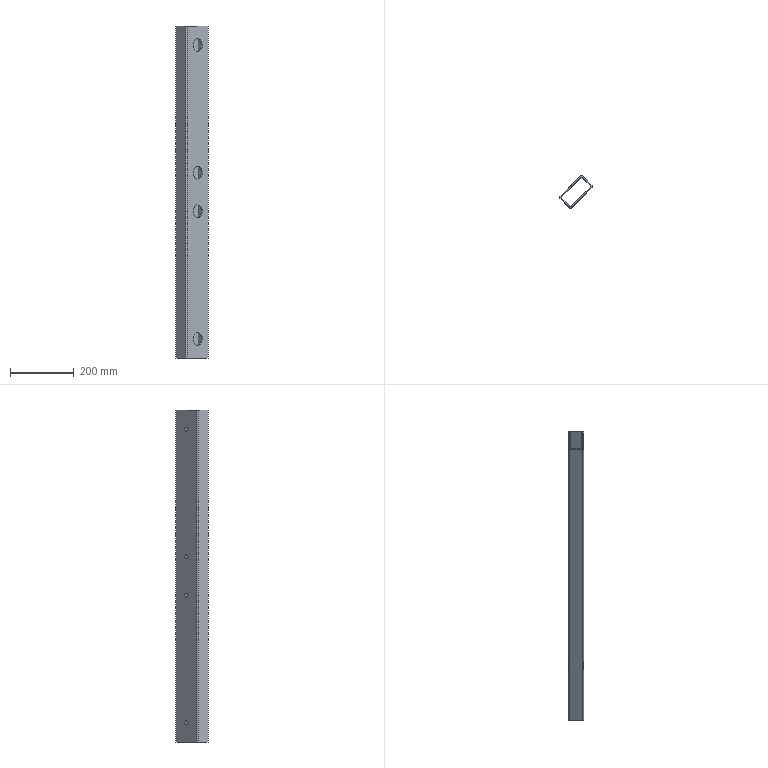Component | NX | VERTICAL_BRACKET_CONN_BEAM | 1 solid | 26 faces | volume 1158192 mm3 | cylinder 16 | plane 10 | commonest cylinder face diameters 8 x8 13 x4 41 x4